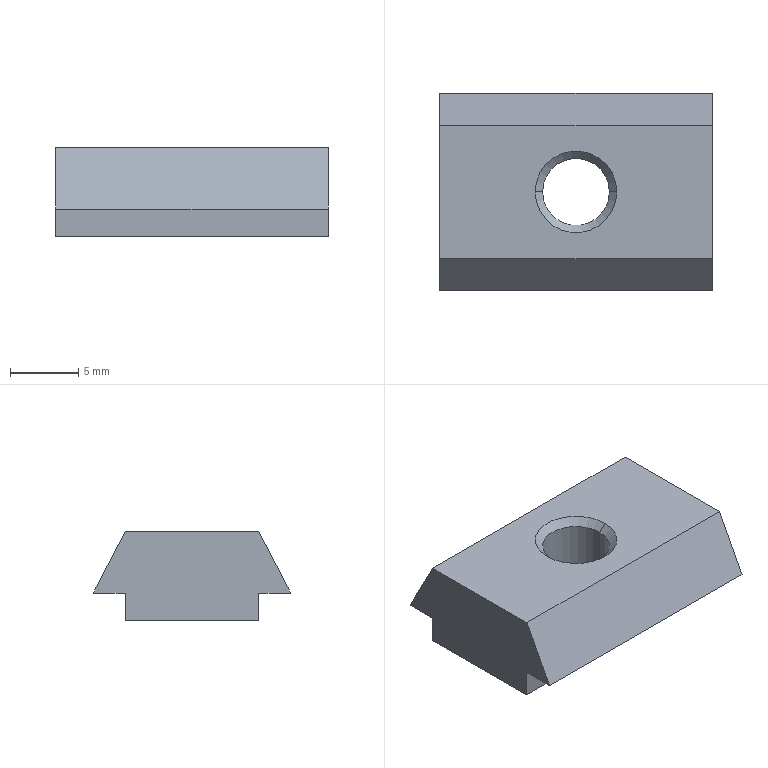Component | SolidWorks | Q1-A12-S21-Q1A.SLDASQ-1_Q1-HNTA8-6-2 | 1 solid | 16 faces | box 20 x 14.5 x 6.5 mm | volume 1357 mm3 | plane 10 | cone 4 | cylinder 2 | commonest cylinder face diameters 4.917 x2
build123d program:
from build123d import *

# Parameters (mm, degrees)
BOSS_EXTRUDE1_DEPTH      = 10
BOSS_EXTRUDE1_DEPTH_BACK = 10


with BuildPart() as part:
    # Sketch1 → Boss-Extrude1 (new, two sides: drawn at the far end of the back side and taken through both)
    with BuildSketch(Plane.XY.offset(-BOSS_EXTRUDE1_DEPTH_BACK)):
        Polygon((0, -4.9), (4.5, -7.25), (4.5, -4.9), (6.5, -4.9), (6.5, 4.9), (4.5, 4.9), (4.5, 7.25), (0, 4.9), align=None)
    extrude(amount=BOSS_EXTRUDE1_DEPTH + BOSS_EXTRUDE1_DEPTH_BACK)

    # Sketch2 → Cut-Revolve1 (revolve, cut)
    with BuildSketch(Plane.XY, mode=Mode.PRIVATE) as cut_revolve1_sk:
        Polygon((0, 0), (0, 3), (0.5415, 2.458), (5.958, 2.458), (6.5, 3), (6.5, 0), align=None)
    revolve(cut_revolve1_sk.sketch.rotate(Axis((6.5, 0, 0), (-1, 0, 0)), 270), axis=Axis((6.5, 0, 0), (-1, 0, 0)), mode=Mode.SUBTRACT)


solid = part.part

# Placed as in the assembly
solid = solid.moved(Location((73.5, -20, -140), (0, 90, 0)))
STEP:
#1=COLOUR_RGB('',0.7922,0.8196,0.9333);
#2=FILL_AREA_STYLE_COLOUR('',#1);
#3=FILL_AREA_STYLE('',(#2));
#4=SURFACE_STYLE_FILL_AREA(#3);
#5=SURFACE_SIDE_STYLE('',(#4));
#6=SURFACE_STYLE_USAGE(.BOTH.,#5);
#7=PRESENTATION_STYLE_ASSIGNMENT((#6));
#8=CARTESIAN_POINT('',(2.797,-0.7874,-5.746));
#9=VERTEX_POINT('',#8);
#10=CARTESIAN_POINT('',(2.99,-0.7874,-5.746));
#11=VERTEX_POINT('',#10);
#12=CARTESIAN_POINT('',(2.894,-0.7874,-5.746));
#13=DIRECTION('',(0.,-0.,1.));
#14=DIRECTION('',(1.,0.,0.));
#15=AXIS2_PLACEMENT_3D('',#12,#13,#14);
#16=CIRCLE('',#15,0.09679);
#17=EDGE_CURVE('',#9,#11,#16,.T.);
#18=ORIENTED_EDGE('',*,*,#17,.T.);
#19=CARTESIAN_POINT('',(3.012,-0.7874,-5.768));
#20=VERTEX_POINT('',#19);
#21=CARTESIAN_POINT('',(3.012,-0.7874,-5.768));
#22=DIRECTION('',(0.7071,0.,-0.7071));
#23=VECTOR('',#22,39.37);
#24=LINE('',#21,#23);
#25=EDGE_CURVE('',#11,#20,#24,.T.);
#26=ORIENTED_EDGE('',*,*,#25,.T.);
#27=CARTESIAN_POINT('',(2.776,-0.7874,-5.768));
#28=VERTEX_POINT('',#27);
#29=CARTESIAN_POINT('',(2.894,-0.7874,-5.768));
#30=DIRECTION('',(0.,-0.,1.));
#31=DIRECTION('',(1.,0.,0.));
#32=AXIS2_PLACEMENT_3D('',#29,#30,#31);
#33=CIRCLE('',#32,0.1181);
#34=EDGE_CURVE('',#28,#20,#33,.T.);
#35=ORIENTED_EDGE('',*,*,#34,.F.);
#36=CARTESIAN_POINT('',(2.776,-0.7874,-5.768));
#37=DIRECTION('',(-0.7071,0.,-0.7071));
#38=VECTOR('',#37,39.37);
#39=LINE('',#36,#38);
#40=EDGE_CURVE('',#9,#28,#39,.T.);
#41=ORIENTED_EDGE('',*,*,#40,.F.);
#42=EDGE_LOOP('',(#18,#26,#35,#41));
#43=FACE_OUTER_BOUND('',#42,.T.);
#44=CARTESIAN_POINT('',(2.894,-0.7874,-5.768));
#45=DIRECTION('',(-0.,0.,-1.));
#46=DIRECTION('',(-1.,0.,0.));
#47=AXIS2_PLACEMENT_3D('',#44,#45,#46);
#48=CONICAL_SURFACE('',#47,0.1181,0.7854);
#49=ADVANCED_FACE('',(#43),#48,.F.);
#50=ORIENTED_EDGE('',*,*,#17,.F.);
#51=CARTESIAN_POINT('',(2.797,-0.7874,-5.533));
#52=VERTEX_POINT('',#51);
#53=CARTESIAN_POINT('',(2.797,-0.7874,-5.768));
#54=DIRECTION('',(0.,-0.,1.));
#55=VECTOR('',#54,39.37);
#56=LINE('',#53,#55);
#57=EDGE_CURVE('',#9,#52,#56,.T.);
#58=ORIENTED_EDGE('',*,*,#57,.T.);
#59=CARTESIAN_POINT('',(2.99,-0.7874,-5.533));
#60=VERTEX_POINT('',#59);
#61=CARTESIAN_POINT('',(2.894,-0.7874,-5.533));
#62=DIRECTION('',(0.,-0.,1.));
#63=DIRECTION('',(1.,0.,0.));
#64=AXIS2_PLACEMENT_3D('',#61,#62,#63);
#65=CIRCLE('',#64,0.09679);
#66=EDGE_CURVE('',#52,#60,#65,.T.);
#67=ORIENTED_EDGE('',*,*,#66,.T.);
#68=CARTESIAN_POINT('',(2.99,-0.7874,-5.768));
#69=DIRECTION('',(0.,-0.,1.));
#70=VECTOR('',#69,39.37);
#71=LINE('',#68,#70);
#72=EDGE_CURVE('',#11,#60,#71,.T.);
#73=ORIENTED_EDGE('',*,*,#72,.F.);
#74=EDGE_LOOP('',(#50,#58,#67,#73));
#75=FACE_OUTER_BOUND('',#74,.T.);
#76=CARTESIAN_POINT('',(2.894,-0.7874,-5.768));
#77=DIRECTION('',(0.,-0.,1.));
#78=DIRECTION('',(1.,0.,0.));
#79=AXIS2_PLACEMENT_3D('',#76,#77,#78);
#80=CYLINDRICAL_SURFACE('',#79,0.09679);
#81=ADVANCED_FACE('',(#75),#80,.F.);
#82=ORIENTED_EDGE('',*,*,#66,.F.);
#83=CARTESIAN_POINT('',(2.776,-0.7874,-5.512));
#84=VERTEX_POINT('',#83);
#85=CARTESIAN_POINT('',(2.797,-0.7874,-5.533));
#86=DIRECTION('',(-0.7071,0.,0.7071));
#87=VECTOR('',#86,39.37);
#88=LINE('',#85,#87);
#89=EDGE_CURVE('',#52,#84,#88,.T.);
#90=ORIENTED_EDGE('',*,*,#89,.T.);
#91=CARTESIAN_POINT('',(3.012,-0.7874,-5.512));
#92=VERTEX_POINT('',#91);
#93=CARTESIAN_POINT('',(2.894,-0.7874,-5.512));
#94=DIRECTION('',(0.,-0.,1.));
#95=DIRECTION('',(1.,0.,0.));
#96=AXIS2_PLACEMENT_3D('',#93,#94,#95);
#97=CIRCLE('',#96,0.1181);
#98=EDGE_CURVE('',#84,#92,#97,.T.);
#99=ORIENTED_EDGE('',*,*,#98,.T.);
#100=CARTESIAN_POINT('',(2.99,-0.7874,-5.533));
#101=DIRECTION('',(0.7071,-0.,0.7071));
#102=VECTOR('',#101,39.37);
#103=LINE('',#100,#102);
#104=EDGE_CURVE('',#60,#92,#103,.T.);
#105=ORIENTED_EDGE('',*,*,#104,.F.);
#106=EDGE_LOOP('',(#82,#90,#99,#105));
#107=FACE_OUTER_BOUND('',#106,.T.);
#108=CARTESIAN_POINT('',(2.894,-0.7874,-5.533));
#109=DIRECTION('',(0.,-0.,1.));
#110=DIRECTION('',(1.,0.,0.));
#111=AXIS2_PLACEMENT_3D('',#108,#109,#110);
#112=CONICAL_SURFACE('',#111,0.09679,0.7854);
#113=ADVANCED_FACE('',(#107),#112,.F.);
#114=CARTESIAN_POINT('',(2.894,-0.7874,-5.512));
#115=DIRECTION('',(0.,-0.,1.));
#116=DIRECTION('',(1.,0.,0.));
#117=AXIS2_PLACEMENT_3D('',#114,#115,#116);
#118=CIRCLE('',#117,0.1181);
#119=EDGE_CURVE('',#92,#84,#118,.T.);
#120=ORIENTED_EDGE('',*,*,#119,.F.);
#121=ORIENTED_EDGE('',*,*,#98,.F.);
#122=EDGE_LOOP('',(#120,#121));
#123=FACE_BOUND('',#122,.T.);
#124=CARTESIAN_POINT('',(3.287,-0.5945,-5.512));
#125=VERTEX_POINT('',#124);
#126=CARTESIAN_POINT('',(2.5,-0.5945,-5.512));
#127=VERTEX_POINT('',#126);
#128=CARTESIAN_POINT('',(3.287,-0.5945,-5.512));
#129=DIRECTION('',(-1.,0.,0.));
#130=VECTOR('',#129,39.37);
#131=LINE('',#128,#130);
#132=EDGE_CURVE('',#125,#127,#131,.T.);
#133=ORIENTED_EDGE('',*,*,#132,.T.);
#134=CARTESIAN_POINT('',(2.5,-0.9803,-5.512));
#135=VERTEX_POINT('',#134);
#136=CARTESIAN_POINT('',(2.5,-0.5945,-5.512));
#137=DIRECTION('',(0.,-1.,-0.));
#138=VECTOR('',#137,39.37);
#139=LINE('',#136,#138);
#140=EDGE_CURVE('',#127,#135,#139,.T.);
#141=ORIENTED_EDGE('',*,*,#140,.T.);
#142=CARTESIAN_POINT('',(3.287,-0.9803,-5.512));
#143=VERTEX_POINT('',#142);
#144=CARTESIAN_POINT('',(3.287,-0.9803,-5.512));
#145=DIRECTION('',(-1.,0.,0.));
#146=VECTOR('',#145,39.37);
#147=LINE('',#144,#146);
#148=EDGE_CURVE('',#143,#135,#147,.T.);
#149=ORIENTED_EDGE('',*,*,#148,.F.);
#150=CARTESIAN_POINT('',(3.287,-0.5945,-5.512));
#151=DIRECTION('',(0.,-1.,-0.));
#152=VECTOR('',#151,39.37);
#153=LINE('',#150,#152);
#154=EDGE_CURVE('',#125,#143,#153,.T.);
#155=ORIENTED_EDGE('',*,*,#154,.F.);
#156=EDGE_LOOP('',(#133,#141,#149,#155));
#157=FACE_OUTER_BOUND('',#156,.T.);
#158=CARTESIAN_POINT('',(3.287,-0.5945,-5.512));
#159=DIRECTION('',(-0.,0.,-1.));
#160=DIRECTION('',(-1.,0.,0.));
#161=AXIS2_PLACEMENT_3D('',#158,#159,#160);
#162=PLANE('',#161);
#163=ADVANCED_FACE('',(#123,#157),#162,.F.);
#164=ORIENTED_EDGE('',*,*,#148,.T.);
#165=CARTESIAN_POINT('',(2.5,-1.073,-5.689));
#166=VERTEX_POINT('',#165);
#167=CARTESIAN_POINT('',(2.5,-0.9803,-5.512));
#168=DIRECTION('',(-0.,-0.4629,-0.8864));
#169=VECTOR('',#168,39.37);
#170=LINE('',#167,#169);
#171=EDGE_CURVE('',#135,#166,#170,.T.);
#172=ORIENTED_EDGE('',*,*,#171,.T.);
#173=CARTESIAN_POINT('',(3.287,-1.073,-5.689));
#174=VERTEX_POINT('',#173);
#175=CARTESIAN_POINT('',(3.287,-1.073,-5.689));
#176=DIRECTION('',(-1.,0.,0.));
#177=VECTOR('',#176,39.37);
#178=LINE('',#175,#177);
#179=EDGE_CURVE('',#174,#166,#178,.T.);
#180=ORIENTED_EDGE('',*,*,#179,.F.);
#181=CARTESIAN_POINT('',(3.287,-0.9803,-5.512));
#182=DIRECTION('',(-0.,-0.4629,-0.8864));
#183=VECTOR('',#182,39.37);
#184=LINE('',#181,#183);
#185=EDGE_CURVE('',#143,#174,#184,.T.);
#186=ORIENTED_EDGE('',*,*,#185,.F.);
#187=EDGE_LOOP('',(#164,#172,#180,#186));
#188=FACE_OUTER_BOUND('',#187,.T.);
#189=CARTESIAN_POINT('',(3.287,-0.9803,-5.512));
#190=DIRECTION('',(-0.,0.8864,-0.4629));
#191=DIRECTION('',(0.,0.4629,0.8864));
#192=AXIS2_PLACEMENT_3D('',#189,#190,#191);
#193=PLANE('',#192);
#194=ADVANCED_FACE('',(#188),#193,.F.);
#195=ORIENTED_EDGE('',*,*,#179,.T.);
#196=CARTESIAN_POINT('',(2.5,-0.9803,-5.689));
#197=VERTEX_POINT('',#196);
#198=CARTESIAN_POINT('',(2.5,-1.073,-5.689));
#199=DIRECTION('',(-0.,1.,0.));
#200=VECTOR('',#199,39.37);
#201=LINE('',#198,#200);
#202=EDGE_CURVE('',#166,#197,#201,.T.);
#203=ORIENTED_EDGE('',*,*,#202,.T.);
#204=CARTESIAN_POINT('',(3.287,-0.9803,-5.689));
#205=VERTEX_POINT('',#204);
#206=CARTESIAN_POINT('',(3.287,-0.9803,-5.689));
#207=DIRECTION('',(-1.,0.,0.));
#208=VECTOR('',#207,39.37);
#209=LINE('',#206,#208);
#210=EDGE_CURVE('',#205,#197,#209,.T.);
#211=ORIENTED_EDGE('',*,*,#210,.F.);
#212=CARTESIAN_POINT('',(3.287,-1.073,-5.689));
#213=DIRECTION('',(-0.,1.,0.));
#214=VECTOR('',#213,39.37);
#215=LINE('',#212,#214);
#216=EDGE_CURVE('',#174,#205,#215,.T.);
#217=ORIENTED_EDGE('',*,*,#216,.F.);
#218=EDGE_LOOP('',(#195,#203,#211,#217));
#219=FACE_OUTER_BOUND('',#218,.T.);
#220=CARTESIAN_POINT('',(3.287,-1.073,-5.689));
#221=DIRECTION('',(0.,-0.,1.));
#222=DIRECTION('',(1.,-0.,-0.));
#223=AXIS2_PLACEMENT_3D('',#220,#221,#222);
#224=PLANE('',#223);
#225=ADVANCED_FACE('',(#219),#224,.F.);
#226=ORIENTED_EDGE('',*,*,#210,.T.);
#227=CARTESIAN_POINT('',(2.5,-0.9803,-5.768));
#228=VERTEX_POINT('',#227);
#229=CARTESIAN_POINT('',(2.5,-0.9803,-5.689));
#230=DIRECTION('',(-0.,0.,-1.));
#231=VECTOR('',#230,39.37);
#232=LINE('',#229,#231);
#233=EDGE_CURVE('',#197,#228,#232,.T.);
#234=ORIENTED_EDGE('',*,*,#233,.T.);
#235=CARTESIAN_POINT('',(3.287,-0.9803,-5.768));
#236=VERTEX_POINT('',#235);
#237=CARTESIAN_POINT('',(3.287,-0.9803,-5.768));
#238=DIRECTION('',(-1.,0.,0.));
#239=VECTOR('',#238,39.37);
#240=LINE('',#237,#239);
#241=EDGE_CURVE('',#236,#228,#240,.T.);
#242=ORIENTED_EDGE('',*,*,#241,.F.);
#243=CARTESIAN_POINT('',(3.287,-0.9803,-5.689));
#244=DIRECTION('',(-0.,0.,-1.));
#245=VECTOR('',#244,39.37);
#246=LINE('',#243,#245);
#247=EDGE_CURVE('',#205,#236,#246,.T.);
#248=ORIENTED_EDGE('',*,*,#247,.F.);
#249=EDGE_LOOP('',(#226,#234,#242,#248));
#250=FACE_OUTER_BOUND('',#249,.T.);
#251=CARTESIAN_POINT('',(3.287,-0.9803,-5.689));
#252=DIRECTION('',(0.,1.,0.));
#253=DIRECTION('',(1.,-0.,-0.));
#254=AXIS2_PLACEMENT_3D('',#251,#252,#253);
#255=PLANE('',#254);
#256=ADVANCED_FACE('',(#250),#255,.F.);
#257=ORIENTED_EDGE('',*,*,#34,.T.);
#258=CARTESIAN_POINT('',(2.894,-0.7874,-5.768));
#259=DIRECTION('',(0.,-0.,1.));
#260=DIRECTION('',(1.,0.,0.));
#261=AXIS2_PLACEMENT_3D('',#258,#259,#260);
#262=CIRCLE('',#261,0.1181);
#263=EDGE_CURVE('',#20,#28,#262,.T.);
#264=ORIENTED_EDGE('',*,*,#263,.T.);
#265=EDGE_LOOP('',(#257,#264));
#266=FACE_BOUND('',#265,.T.);
#267=ORIENTED_EDGE('',*,*,#241,.T.);
#268=CARTESIAN_POINT('',(2.5,-0.5945,-5.768));
#269=VERTEX_POINT('',#268);
#270=CARTESIAN_POINT('',(2.5,-0.9803,-5.768));
#271=DIRECTION('',(-0.,1.,0.));
#272=VECTOR('',#271,39.37);
#273=LINE('',#270,#272);
#274=EDGE_CURVE('',#228,#269,#273,.T.);
#275=ORIENTED_EDGE('',*,*,#274,.T.);
#276=CARTESIAN_POINT('',(3.287,-0.5945,-5.768));
#277=VERTEX_POINT('',#276);
#278=CARTESIAN_POINT('',(3.287,-0.5945,-5.768));
#279=DIRECTION('',(-1.,0.,0.));
#280=VECTOR('',#279,39.37);
#281=LINE('',#278,#280);
#282=EDGE_CURVE('',#277,#269,#281,.T.);
#283=ORIENTED_EDGE('',*,*,#282,.F.);
#284=CARTESIAN_POINT('',(3.287,-0.9803,-5.768));
#285=DIRECTION('',(-0.,1.,0.));
#286=VECTOR('',#285,39.37);
#287=LINE('',#284,#286);
#288=EDGE_CURVE('',#236,#277,#287,.T.);
#289=ORIENTED_EDGE('',*,*,#288,.F.);
#290=EDGE_LOOP('',(#267,#275,#283,#289));
#291=FACE_OUTER_BOUND('',#290,.T.);
#292=CARTESIAN_POINT('',(3.287,-0.9803,-5.768));
#293=DIRECTION('',(0.,-0.,1.));
#294=DIRECTION('',(1.,-0.,-0.));
#295=AXIS2_PLACEMENT_3D('',#292,#293,#294);
#296=PLANE('',#295);
#297=ADVANCED_FACE('',(#266,#291),#296,.F.);
#298=ORIENTED_EDGE('',*,*,#282,.T.);
#299=CARTESIAN_POINT('',(2.5,-0.5945,-5.689));
#300=VERTEX_POINT('',#299);
#301=CARTESIAN_POINT('',(2.5,-0.5945,-5.768));
#302=DIRECTION('',(0.,-0.,1.));
#303=VECTOR('',#302,39.37);
#304=LINE('',#301,#303);
#305=EDGE_CURVE('',#269,#300,#304,.T.);
#306=ORIENTED_EDGE('',*,*,#305,.T.);
#307=CARTESIAN_POINT('',(3.287,-0.5945,-5.689));
#308=VERTEX_POINT('',#307);
#309=CARTESIAN_POINT('',(3.287,-0.5945,-5.689));
#310=DIRECTION('',(-1.,0.,0.));
#311=VECTOR('',#310,39.37);
#312=LINE('',#309,#311);
#313=EDGE_CURVE('',#308,#300,#312,.T.);
#314=ORIENTED_EDGE('',*,*,#313,.F.);
#315=CARTESIAN_POINT('',(3.287,-0.5945,-5.768));
#316=DIRECTION('',(0.,-0.,1.));
#317=VECTOR('',#316,39.37);
#318=LINE('',#315,#317);
#319=EDGE_CURVE('',#277,#308,#318,.T.);
#320=ORIENTED_EDGE('',*,*,#319,.F.);
#321=EDGE_LOOP('',(#298,#306,#314,#320));
#322=FACE_OUTER_BOUND('',#321,.T.);
#323=CARTESIAN_POINT('',(3.287,-0.5945,-5.768));
#324=DIRECTION('',(-0.,-1.,-0.));
#325=DIRECTION('',(-1.,0.,0.));
#326=AXIS2_PLACEMENT_3D('',#323,#324,#325);
#327=PLANE('',#326);
#328=ADVANCED_FACE('',(#322),#327,.F.);
#329=ORIENTED_EDGE('',*,*,#313,.T.);
#330=CARTESIAN_POINT('',(2.5,-0.502,-5.689));
#331=VERTEX_POINT('',#330);
#332=CARTESIAN_POINT('',(2.5,-0.5945,-5.689));
#333=DIRECTION('',(-0.,1.,0.));
#334=VECTOR('',#333,39.37);
#335=LINE('',#332,#334);
#336=EDGE_CURVE('',#300,#331,#335,.T.);
#337=ORIENTED_EDGE('',*,*,#336,.T.);
#338=CARTESIAN_POINT('',(3.287,-0.502,-5.689));
#339=VERTEX_POINT('',#338);
#340=CARTESIAN_POINT('',(3.287,-0.502,-5.689));
#341=DIRECTION('',(-1.,0.,0.));
#342=VECTOR('',#341,39.37);
#343=LINE('',#340,#342);
#344=EDGE_CURVE('',#339,#331,#343,.T.);
#345=ORIENTED_EDGE('',*,*,#344,.F.);
#346=CARTESIAN_POINT('',(3.287,-0.5945,-5.689));
#347=DIRECTION('',(-0.,1.,0.));
#348=VECTOR('',#347,39.37);
#349=LINE('',#346,#348);
#350=EDGE_CURVE('',#308,#339,#349,.T.);
#351=ORIENTED_EDGE('',*,*,#350,.F.);
#352=EDGE_LOOP('',(#329,#337,#345,#351));
#353=FACE_OUTER_BOUND('',#352,.T.);
#354=CARTESIAN_POINT('',(3.287,-0.5945,-5.689));
#355=DIRECTION('',(0.,-0.,1.));
#356=DIRECTION('',(1.,-0.,-0.));
#357=AXIS2_PLACEMENT_3D('',#354,#355,#356);
#358=PLANE('',#357);
#359=ADVANCED_FACE('',(#353),#358,.F.);
#360=ORIENTED_EDGE('',*,*,#344,.T.);
#361=CARTESIAN_POINT('',(2.5,-0.502,-5.689));
#362=DIRECTION('',(0.,-0.4629,0.8864));
#363=VECTOR('',#362,39.37);
#364=LINE('',#361,#363);
#365=EDGE_CURVE('',#331,#127,#364,.T.);
#366=ORIENTED_EDGE('',*,*,#365,.T.);
#367=ORIENTED_EDGE('',*,*,#132,.F.);
#368=CARTESIAN_POINT('',(3.287,-0.502,-5.689));
#369=DIRECTION('',(0.,-0.4629,0.8864));
#370=VECTOR('',#369,39.37);
#371=LINE('',#368,#370);
#372=EDGE_CURVE('',#339,#125,#371,.T.);
#373=ORIENTED_EDGE('',*,*,#372,.F.);
#374=EDGE_LOOP('',(#360,#366,#367,#373));
#375=FACE_OUTER_BOUND('',#374,.T.);
#376=CARTESIAN_POINT('',(3.287,-0.502,-5.689));
#377=DIRECTION('',(0.,-0.8864,-0.4629));
#378=DIRECTION('',(-0.,0.4629,-0.8864));
#379=AXIS2_PLACEMENT_3D('',#376,#377,#378);
#380=PLANE('',#379);
#381=ADVANCED_FACE('',(#375),#380,.F.);
#382=ORIENTED_EDGE('',*,*,#154,.T.);
#383=ORIENTED_EDGE('',*,*,#185,.T.);
#384=ORIENTED_EDGE('',*,*,#216,.T.);
#385=ORIENTED_EDGE('',*,*,#247,.T.);
#386=ORIENTED_EDGE('',*,*,#288,.T.);
#387=ORIENTED_EDGE('',*,*,#319,.T.);
#388=ORIENTED_EDGE('',*,*,#350,.T.);
#389=ORIENTED_EDGE('',*,*,#372,.T.);
#390=EDGE_LOOP('',(#382,#383,#384,#385,#386,#387,#388,#389));
#391=FACE_OUTER_BOUND('',#390,.T.);
#392=CARTESIAN_POINT('',(3.287,-0.7874,-5.512));
#393=DIRECTION('',(1.,-0.,-0.));
#394=DIRECTION('',(-0.,0.,-1.));
#395=AXIS2_PLACEMENT_3D('',#392,#393,#394);
#396=PLANE('',#395);
#397=ADVANCED_FACE('',(#391),#396,.T.);
#398=ORIENTED_EDGE('',*,*,#140,.F.);
#399=ORIENTED_EDGE('',*,*,#365,.F.);
#400=ORIENTED_EDGE('',*,*,#336,.F.);
#401=ORIENTED_EDGE('',*,*,#305,.F.);
#402=ORIENTED_EDGE('',*,*,#274,.F.);
#403=ORIENTED_EDGE('',*,*,#233,.F.);
#404=ORIENTED_EDGE('',*,*,#202,.F.);
#405=ORIENTED_EDGE('',*,*,#171,.F.);
#406=EDGE_LOOP('',(#398,#399,#400,#401,#402,#403,#404,#405));
#407=FACE_OUTER_BOUND('',#406,.T.);
#408=CARTESIAN_POINT('',(2.5,-0.7874,-5.512));
#409=DIRECTION('',(1.,-0.,-0.));
#410=DIRECTION('',(-0.,0.,-1.));
#411=AXIS2_PLACEMENT_3D('',#408,#409,#410);
#412=PLANE('',#411);
#413=ADVANCED_FACE('',(#407),#412,.F.);
#414=ORIENTED_EDGE('',*,*,#89,.F.);
#415=CARTESIAN_POINT('',(2.894,-0.7874,-5.533));
#416=DIRECTION('',(0.,-0.,1.));
#417=DIRECTION('',(1.,0.,0.));
#418=AXIS2_PLACEMENT_3D('',#415,#416,#417);
#419=CIRCLE('',#418,0.09679);
#420=EDGE_CURVE('',#60,#52,#419,.T.);
#421=ORIENTED_EDGE('',*,*,#420,.F.);
#422=ORIENTED_EDGE('',*,*,#104,.T.);
#423=ORIENTED_EDGE('',*,*,#119,.T.);
#424=EDGE_LOOP('',(#414,#421,#422,#423));
#425=FACE_OUTER_BOUND('',#424,.T.);
#426=CARTESIAN_POINT('',(2.894,-0.7874,-5.533));
#427=DIRECTION('',(0.,-0.,1.));
#428=DIRECTION('',(1.,0.,0.));
#429=AXIS2_PLACEMENT_3D('',#426,#427,#428);
#430=CONICAL_SURFACE('',#429,0.09679,0.7854);
#431=ADVANCED_FACE('',(#425),#430,.F.);
#432=ORIENTED_EDGE('',*,*,#57,.F.);
#433=CARTESIAN_POINT('',(2.894,-0.7874,-5.746));
#434=DIRECTION('',(0.,-0.,1.));
#435=DIRECTION('',(1.,0.,0.));
#436=AXIS2_PLACEMENT_3D('',#433,#434,#435);
#437=CIRCLE('',#436,0.09679);
#438=EDGE_CURVE('',#11,#9,#437,.T.);
#439=ORIENTED_EDGE('',*,*,#438,.F.);
#440=ORIENTED_EDGE('',*,*,#72,.T.);
#441=ORIENTED_EDGE('',*,*,#420,.T.);
#442=EDGE_LOOP('',(#432,#439,#440,#441));
#443=FACE_OUTER_BOUND('',#442,.T.);
#444=CARTESIAN_POINT('',(2.894,-0.7874,-5.768));
#445=DIRECTION('',(0.,-0.,1.));
#446=DIRECTION('',(1.,0.,0.));
#447=AXIS2_PLACEMENT_3D('',#444,#445,#446);
#448=CYLINDRICAL_SURFACE('',#447,0.09679);
#449=ADVANCED_FACE('',(#443),#448,.F.);
#450=ORIENTED_EDGE('',*,*,#25,.F.);
#451=ORIENTED_EDGE('',*,*,#438,.T.);
#452=ORIENTED_EDGE('',*,*,#40,.T.);
#453=ORIENTED_EDGE('',*,*,#263,.F.);
#454=EDGE_LOOP('',(#450,#451,#452,#453));
#455=FACE_OUTER_BOUND('',#454,.T.);
#456=CARTESIAN_POINT('',(2.894,-0.7874,-5.768));
#457=DIRECTION('',(-0.,0.,-1.));
#458=DIRECTION('',(-1.,0.,0.));
#459=AXIS2_PLACEMENT_3D('',#456,#457,#458);
#460=CONICAL_SURFACE('',#459,0.1181,0.7854);
#461=ADVANCED_FACE('',(#455),#460,.F.);
#462=CLOSED_SHELL('',(#49,#81,#113,#163,#194,#225,#256,#297,#328,#359,#381,#397,#413,#431,#449,#461));
#463=MANIFOLD_SOLID_BREP('',#462);
#464=STYLED_ITEM('',(#7),#463);
#465=(LENGTH_UNIT()NAMED_UNIT(*)SI_UNIT($,.METRE.));
#466=LENGTH_MEASURE_WITH_UNIT(LENGTH_MEASURE(0.0254),#465);
#467=DIMENSIONAL_EXPONENTS(1.,0.,0.,0.,0.,0.,0.);
#468=(CONVERSION_BASED_UNIT('',#466)LENGTH_UNIT()NAMED_UNIT(#467));
#469=UNCERTAINTY_MEASURE_WITH_UNIT(LENGTH_MEASURE(0.00001),#468,'','');
#470=(NAMED_UNIT(*)PLANE_ANGLE_UNIT()SI_UNIT($,.RADIAN.));
#471=(NAMED_UNIT(*)SI_UNIT($,.STERADIAN.)SOLID_ANGLE_UNIT());
#472=(GEOMETRIC_REPRESENTATION_CONTEXT(3)GLOBAL_UNCERTAINTY_ASSIGNED_CONTEXT((#469))GLOBAL_UNIT_ASSIGNED_CONTEXT((#468,#470,#471))REPRESENTATION_CONTEXT('',''));
#473=MECHANICAL_DESIGN_GEOMETRIC_PRESENTATION_REPRESENTATION('',(#464),#472);
#474=PRESENTATION_LAYER_ASSIGNMENT('','',(#464));
#475=CARTESIAN_POINT('',(0.,0.,0.));
#476=DIRECTION('',(0.,0.,1.));
#477=DIRECTION('',(1.,0.,0.));
#478=AXIS2_PLACEMENT_3D('',#475,#476,#477);
#479=(LENGTH_UNIT()NAMED_UNIT(*)SI_UNIT($,.METRE.));
#480=LENGTH_MEASURE_WITH_UNIT(LENGTH_MEASURE(0.0254),#479);
#481=DIMENSIONAL_EXPONENTS(1.,0.,0.,0.,0.,0.,0.);
#482=(CONVERSION_BASED_UNIT('',#480)LENGTH_UNIT()NAMED_UNIT(#481));
#483=UNCERTAINTY_MEASURE_WITH_UNIT(LENGTH_MEASURE(0.00001),#482,'','');
#484=(NAMED_UNIT(*)PLANE_ANGLE_UNIT()SI_UNIT($,.RADIAN.));
#485=(NAMED_UNIT(*)SI_UNIT($,.STERADIAN.)SOLID_ANGLE_UNIT());
#486=(GEOMETRIC_REPRESENTATION_CONTEXT(3)GLOBAL_UNCERTAINTY_ASSIGNED_CONTEXT((#483))GLOBAL_UNIT_ASSIGNED_CONTEXT((#482,#484,#485))REPRESENTATION_CONTEXT('',''));
#487=ADVANCED_BREP_SHAPE_REPRESENTATION('',(#463,#478),#486);